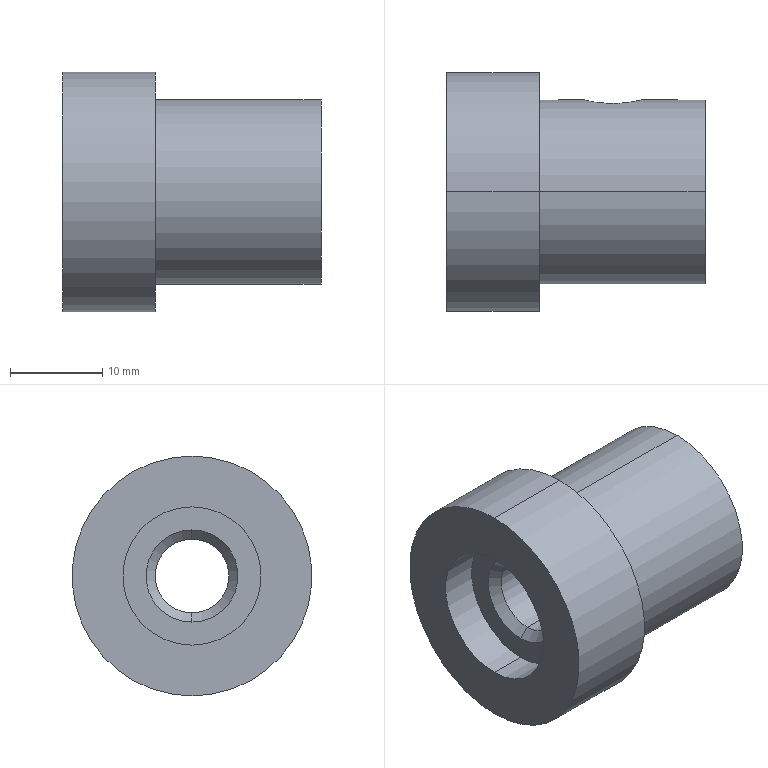Component | SolidWorks | LongAxisUpperSleeve-1 | 1 solid | 18 faces | box 28 x 26 x 26 mm | volume 8975 mm3 | cylinder 10 | cone 4 | plane 4 | commonest cylinder face diameters 3.2 x2 26 x2 20 x2 8 x2 15 x2 | material 5154-O, Bar (SS)
STEP:
#1=COLOUR_RGB('',0.7922,0.8196,0.9333);
#2=FILL_AREA_STYLE_COLOUR('',#1);
#3=FILL_AREA_STYLE('',(#2));
#4=SURFACE_STYLE_FILL_AREA(#3);
#5=SURFACE_SIDE_STYLE('',(#4));
#6=SURFACE_STYLE_USAGE(.BOTH.,#5);
#7=PRESENTATION_STYLE_ASSIGNMENT((#6));
#8=CARTESIAN_POINT('',(3.546,0.7394,13.677));
#9=VERTEX_POINT('',#8);
#10=CARTESIAN_POINT('',(3.546,0.7394,13.803));
#11=VERTEX_POINT('',#10);
#12=CARTESIAN_POINT('',(3.546,0.7394,13.677));
#13=CARTESIAN_POINT('',(3.542,0.7394,13.677));
#14=CARTESIAN_POINT('',(3.537,0.7396,13.678));
#15=CARTESIAN_POINT('',(3.529,0.7403,13.679));
#16=CARTESIAN_POINT('',(3.525,0.7408,13.68));
#17=CARTESIAN_POINT('',(3.514,0.7427,13.685));
#18=CARTESIAN_POINT('',(3.507,0.7444,13.69));
#19=CARTESIAN_POINT('',(3.498,0.747,13.699));
#20=CARTESIAN_POINT('',(3.496,0.7478,13.702));
#21=CARTESIAN_POINT('',(3.491,0.7494,13.708));
#22=CARTESIAN_POINT('',(3.489,0.7501,13.712));
#23=CARTESIAN_POINT('',(3.486,0.7513,13.72));
#24=CARTESIAN_POINT('',(3.485,0.7518,13.724));
#25=CARTESIAN_POINT('',(3.483,0.7524,13.732));
#26=CARTESIAN_POINT('',(3.483,0.7526,13.736));
#27=CARTESIAN_POINT('',(3.483,0.7526,13.748));
#28=CARTESIAN_POINT('',(3.484,0.7519,13.757));
#29=CARTESIAN_POINT('',(3.489,0.7501,13.768));
#30=CARTESIAN_POINT('',(3.491,0.7494,13.772));
#31=CARTESIAN_POINT('',(3.496,0.7478,13.779));
#32=CARTESIAN_POINT('',(3.498,0.747,13.782));
#33=CARTESIAN_POINT('',(3.504,0.7453,13.788));
#34=CARTESIAN_POINT('',(3.507,0.7444,13.79));
#35=CARTESIAN_POINT('',(3.514,0.7428,13.795));
#36=CARTESIAN_POINT('',(3.518,0.7421,13.797));
#37=CARTESIAN_POINT('',(3.529,0.7402,13.801));
#38=CARTESIAN_POINT('',(3.537,0.7394,13.803));
#39=CARTESIAN_POINT('',(3.546,0.7394,13.803));
#40=B_SPLINE_CURVE_WITH_KNOTS('',3,(#12,#13,#14,#15,#16,#17,#18,#19,#20,#21,#22,#23,#24,#25,#26,#27,#28,#29,#30,#31,#32,#33,#34,#35,#36,#37,#38,#39),.UNSPECIFIED.,.F.,.F.,(4,2,2,2,2,2,2,2,2,2,2,2,2,4),(0.005056,0.005371,0.005687,0.006318,0.006634,0.00695,0.007265,0.007581,0.008212,0.008528,0.008844,0.009159,0.009475,0.01011),.UNSPECIFIED.);
#41=EDGE_CURVE('',#9,#11,#40,.T.);
#42=ORIENTED_EDGE('',*,*,#41,.F.);
#43=CARTESIAN_POINT('',(3.546,0.9258,13.677));
#44=VERTEX_POINT('',#43);
#45=CARTESIAN_POINT('',(3.546,0.9888,13.677));
#46=DIRECTION('',(0.,1.,0.));
#47=VECTOR('',#46,39.37);
#48=LINE('',#45,#47);
#49=EDGE_CURVE('',#9,#44,#48,.T.);
#50=ORIENTED_EDGE('',*,*,#49,.T.);
#51=CARTESIAN_POINT('',(3.546,0.9258,13.803));
#52=VERTEX_POINT('',#51);
#53=CARTESIAN_POINT('',(3.546,0.9258,13.74));
#54=DIRECTION('',(0.,1.,0.));
#55=DIRECTION('',(0.,0.,1.));
#56=AXIS2_PLACEMENT_3D('',#53,#54,#55);
#57=CIRCLE('',#56,0.06299);
#58=EDGE_CURVE('',#44,#52,#57,.T.);
#59=ORIENTED_EDGE('',*,*,#58,.T.);
#60=CARTESIAN_POINT('',(3.546,0.9888,13.803));
#61=DIRECTION('',(0.,1.,0.));
#62=VECTOR('',#61,39.37);
#63=LINE('',#60,#62);
#64=EDGE_CURVE('',#11,#52,#63,.T.);
#65=ORIENTED_EDGE('',*,*,#64,.F.);
#66=EDGE_LOOP('',(#42,#50,#59,#65));
#67=FACE_OUTER_BOUND('',#66,.T.);
#68=CARTESIAN_POINT('',(3.546,0.9888,13.74));
#69=DIRECTION('',(0.,1.,0.));
#70=DIRECTION('',(0.,0.,1.));
#71=AXIS2_PLACEMENT_3D('',#68,#69,#70);
#72=CYLINDRICAL_SURFACE('',#71,0.06299);
#73=ADVANCED_FACE('',(#67),#72,.F.);
#74=ORIENTED_EDGE('',*,*,#58,.F.);
#75=CARTESIAN_POINT('',(3.546,0.9731,13.63));
#76=VERTEX_POINT('',#75);
#77=CARTESIAN_POINT('',(3.546,0.9888,13.614));
#78=DIRECTION('',(0.,0.7071,-0.7071));
#79=VECTOR('',#78,39.37);
#80=LINE('',#77,#79);
#81=EDGE_CURVE('',#44,#76,#80,.T.);
#82=ORIENTED_EDGE('',*,*,#81,.T.);
#83=CARTESIAN_POINT('',(3.546,0.9731,13.85));
#84=VERTEX_POINT('',#83);
#85=CARTESIAN_POINT('',(3.546,0.9731,13.85));
#86=CARTESIAN_POINT('',(3.53,0.9731,13.85));
#87=CARTESIAN_POINT('',(3.515,0.9738,13.848));
#88=CARTESIAN_POINT('',(3.493,0.9759,13.84));
#89=CARTESIAN_POINT('',(3.486,0.9767,13.837));
#90=CARTESIAN_POINT('',(3.472,0.9785,13.83));
#91=CARTESIAN_POINT('',(3.466,0.9795,13.825));
#92=CARTESIAN_POINT('',(3.454,0.9815,13.816));
#93=CARTESIAN_POINT('',(3.448,0.9825,13.81));
#94=CARTESIAN_POINT('',(3.439,0.9845,13.798));
#95=CARTESIAN_POINT('',(3.434,0.9854,13.792));
#96=CARTESIAN_POINT('',(3.427,0.987,13.778));
#97=CARTESIAN_POINT('',(3.424,0.9877,13.771));
#98=CARTESIAN_POINT('',(3.421,0.9886,13.756));
#99=CARTESIAN_POINT('',(3.42,0.9888,13.748));
#100=CARTESIAN_POINT('',(3.42,0.9888,13.732));
#101=CARTESIAN_POINT('',(3.421,0.9886,13.725));
#102=CARTESIAN_POINT('',(3.424,0.9877,13.71));
#103=CARTESIAN_POINT('',(3.427,0.987,13.702));
#104=CARTESIAN_POINT('',(3.434,0.9855,13.689));
#105=CARTESIAN_POINT('',(3.439,0.9845,13.682));
#106=CARTESIAN_POINT('',(3.448,0.9826,13.67));
#107=CARTESIAN_POINT('',(3.454,0.9815,13.665));
#108=CARTESIAN_POINT('',(3.472,0.9784,13.65));
#109=CARTESIAN_POINT('',(3.485,0.9765,13.643));
#110=CARTESIAN_POINT('',(3.507,0.9745,13.635));
#111=CARTESIAN_POINT('',(3.515,0.974,13.633));
#112=CARTESIAN_POINT('',(3.53,0.9732,13.631));
#113=CARTESIAN_POINT('',(3.538,0.9731,13.63));
#114=CARTESIAN_POINT('',(3.546,0.9731,13.63));
#115=B_SPLINE_CURVE_WITH_KNOTS('',3,(#85,#86,#87,#88,#89,#90,#91,#92,#93,#94,#95,#96,#97,#98,#99,#100,#101,#102,#103,#104,#105,#106,#107,#108,#109,#110,#111,#112,#113,#114),.UNSPECIFIED.,.F.,.F.,(4,2,2,2,2,2,2,2,2,2,2,2,2,2,4),(0.01171,0.01289,0.01348,0.01406,0.01465,0.01524,0.01583,0.01642,0.017,0.01759,0.01818,0.01877,0.01994,0.02053,0.02112),.UNSPECIFIED.);
#116=EDGE_CURVE('',#84,#76,#115,.T.);
#117=ORIENTED_EDGE('',*,*,#116,.F.);
#118=CARTESIAN_POINT('',(3.546,0.9888,13.866));
#119=DIRECTION('',(0.,0.7071,0.7071));
#120=VECTOR('',#119,39.37);
#121=LINE('',#118,#120);
#122=EDGE_CURVE('',#52,#84,#121,.T.);
#123=ORIENTED_EDGE('',*,*,#122,.F.);
#124=EDGE_LOOP('',(#74,#82,#117,#123));
#125=FACE_OUTER_BOUND('',#124,.T.);
#126=CARTESIAN_POINT('',(3.546,0.9888,13.74));
#127=DIRECTION('',(0.,1.,0.));
#128=DIRECTION('',(0.,0.,1.));
#129=AXIS2_PLACEMENT_3D('',#126,#127,#128);
#130=CONICAL_SURFACE('',#129,0.126,0.7854);
#131=ADVANCED_FACE('',(#125),#130,.F.);
#132=CARTESIAN_POINT('',(3.231,0.5951,14.252));
#133=VERTEX_POINT('',#132);
#134=CARTESIAN_POINT('',(3.231,0.5951,13.228));
#135=VERTEX_POINT('',#134);
#136=CARTESIAN_POINT('',(3.231,0.5951,13.74));
#137=DIRECTION('',(-1.,0.,0.));
#138=DIRECTION('',(0.,0.,1.));
#139=AXIS2_PLACEMENT_3D('',#136,#137,#138);
#140=CIRCLE('',#139,0.5118);
#141=EDGE_CURVE('',#133,#135,#140,.T.);
#142=ORIENTED_EDGE('',*,*,#141,.T.);
#143=CARTESIAN_POINT('',(2.837,0.5951,13.228));
#144=VERTEX_POINT('',#143);
#145=CARTESIAN_POINT('',(-0.1135,0.5951,13.228));
#146=DIRECTION('',(-1.,0.,0.));
#147=VECTOR('',#146,39.37);
#148=LINE('',#145,#147);
#149=EDGE_CURVE('',#135,#144,#148,.T.);
#150=ORIENTED_EDGE('',*,*,#149,.T.);
#151=CARTESIAN_POINT('',(2.837,0.5951,14.252));
#152=VERTEX_POINT('',#151);
#153=CARTESIAN_POINT('',(2.837,0.5951,13.74));
#154=DIRECTION('',(-1.,0.,0.));
#155=DIRECTION('',(0.,0.,1.));
#156=AXIS2_PLACEMENT_3D('',#153,#154,#155);
#157=CIRCLE('',#156,0.5118);
#158=EDGE_CURVE('',#152,#144,#157,.T.);
#159=ORIENTED_EDGE('',*,*,#158,.F.);
#160=CARTESIAN_POINT('',(-0.1135,0.5951,14.252));
#161=DIRECTION('',(-1.,0.,0.));
#162=VECTOR('',#161,39.37);
#163=LINE('',#160,#162);
#164=EDGE_CURVE('',#133,#152,#163,.T.);
#165=ORIENTED_EDGE('',*,*,#164,.F.);
#166=EDGE_LOOP('',(#142,#150,#159,#165));
#167=FACE_OUTER_BOUND('',#166,.T.);
#168=CARTESIAN_POINT('',(-0.1135,0.5951,13.74));
#169=DIRECTION('',(-1.,0.,0.));
#170=DIRECTION('',(0.,0.,1.));
#171=AXIS2_PLACEMENT_3D('',#168,#169,#170);
#172=CYLINDRICAL_SURFACE('',#171,0.5118);
#173=ADVANCED_FACE('',(#167),#172,.T.);
#174=ORIENTED_EDGE('',*,*,#116,.T.);
#175=CARTESIAN_POINT('',(3.546,0.9731,13.63));
#176=CARTESIAN_POINT('',(3.554,0.9731,13.63));
#177=CARTESIAN_POINT('',(3.561,0.9732,13.631));
#178=CARTESIAN_POINT('',(3.576,0.974,13.633));
#179=CARTESIAN_POINT('',(3.584,0.9745,13.635));
#180=CARTESIAN_POINT('',(3.599,0.9759,13.64));
#181=CARTESIAN_POINT('',(3.606,0.9767,13.643));
#182=CARTESIAN_POINT('',(3.619,0.9785,13.65));
#183=CARTESIAN_POINT('',(3.626,0.9795,13.655));
#184=CARTESIAN_POINT('',(3.638,0.9815,13.665));
#185=CARTESIAN_POINT('',(3.643,0.9825,13.67));
#186=CARTESIAN_POINT('',(3.653,0.9845,13.682));
#187=CARTESIAN_POINT('',(3.657,0.9854,13.688));
#188=CARTESIAN_POINT('',(3.664,0.987,13.702));
#189=CARTESIAN_POINT('',(3.667,0.9877,13.709));
#190=CARTESIAN_POINT('',(3.671,0.9886,13.724));
#191=CARTESIAN_POINT('',(3.672,0.9888,13.732));
#192=CARTESIAN_POINT('',(3.672,0.9888,13.748));
#193=CARTESIAN_POINT('',(3.671,0.9886,13.755));
#194=CARTESIAN_POINT('',(3.667,0.9877,13.77));
#195=CARTESIAN_POINT('',(3.664,0.9871,13.778));
#196=CARTESIAN_POINT('',(3.654,0.9847,13.798));
#197=CARTESIAN_POINT('',(3.644,0.9826,13.811));
#198=CARTESIAN_POINT('',(3.626,0.9795,13.825));
#199=CARTESIAN_POINT('',(3.619,0.9785,13.83));
#200=CARTESIAN_POINT('',(3.606,0.9767,13.837));
#201=CARTESIAN_POINT('',(3.599,0.9759,13.84));
#202=CARTESIAN_POINT('',(3.584,0.9745,13.845));
#203=CARTESIAN_POINT('',(3.577,0.974,13.847));
#204=CARTESIAN_POINT('',(3.561,0.9732,13.85));
#205=CARTESIAN_POINT('',(3.553,0.9731,13.85));
#206=CARTESIAN_POINT('',(3.546,0.9731,13.85));
#207=B_SPLINE_CURVE_WITH_KNOTS('',3,(#175,#176,#177,#178,#179,#180,#181,#182,#183,#184,#185,#186,#187,#188,#189,#190,#191,#192,#193,#194,#195,#196,#197,#198,#199,#200,#201,#202,#203,#204,#205,#206),.UNSPECIFIED.,.F.,.F.,(4,2,2,2,2,2,2,2,2,2,2,2,2,2,2,4),(0.0023,0.002888,0.003477,0.004065,0.004653,0.005242,0.00583,0.006419,0.007007,0.007595,0.008184,0.00936,0.009949,0.01054,0.01113,0.01171),.UNSPECIFIED.);
#208=EDGE_CURVE('',#76,#84,#207,.T.);
#209=ORIENTED_EDGE('',*,*,#208,.T.);
#210=EDGE_LOOP('',(#174,#209));
#211=FACE_BOUND('',#210,.T.);
#212=CARTESIAN_POINT('',(3.939,0.5951,14.134));
#213=VERTEX_POINT('',#212);
#214=CARTESIAN_POINT('',(3.939,0.5951,13.346));
#215=VERTEX_POINT('',#214);
#216=CARTESIAN_POINT('',(3.939,0.5951,13.74));
#217=DIRECTION('',(-1.,0.,0.));
#218=DIRECTION('',(0.,0.,1.));
#219=AXIS2_PLACEMENT_3D('',#216,#217,#218);
#220=CIRCLE('',#219,0.3937);
#221=EDGE_CURVE('',#213,#215,#220,.T.);
#222=ORIENTED_EDGE('',*,*,#221,.T.);
#223=CARTESIAN_POINT('',(3.231,0.5951,13.346));
#224=VERTEX_POINT('',#223);
#225=CARTESIAN_POINT('',(-0.1135,0.5951,13.346));
#226=DIRECTION('',(-1.,0.,0.));
#227=VECTOR('',#226,39.37);
#228=LINE('',#225,#227);
#229=EDGE_CURVE('',#215,#224,#228,.T.);
#230=ORIENTED_EDGE('',*,*,#229,.T.);
#231=CARTESIAN_POINT('',(3.231,0.5951,14.134));
#232=VERTEX_POINT('',#231);
#233=CARTESIAN_POINT('',(3.231,0.5951,13.74));
#234=DIRECTION('',(-1.,0.,0.));
#235=DIRECTION('',(0.,0.,1.));
#236=AXIS2_PLACEMENT_3D('',#233,#234,#235);
#237=CIRCLE('',#236,0.3937);
#238=EDGE_CURVE('',#232,#224,#237,.T.);
#239=ORIENTED_EDGE('',*,*,#238,.F.);
#240=CARTESIAN_POINT('',(-0.1135,0.5951,14.134));
#241=DIRECTION('',(-1.,0.,0.));
#242=VECTOR('',#241,39.37);
#243=LINE('',#240,#242);
#244=EDGE_CURVE('',#213,#232,#243,.T.);
#245=ORIENTED_EDGE('',*,*,#244,.F.);
#246=EDGE_LOOP('',(#222,#230,#239,#245));
#247=FACE_OUTER_BOUND('',#246,.T.);
#248=CARTESIAN_POINT('',(-0.1135,0.5951,13.74));
#249=DIRECTION('',(-1.,0.,0.));
#250=DIRECTION('',(0.,0.,1.));
#251=AXIS2_PLACEMENT_3D('',#248,#249,#250);
#252=CYLINDRICAL_SURFACE('',#251,0.3937);
#253=ADVANCED_FACE('',(#211,#247),#252,.T.);
#254=CARTESIAN_POINT('',(3.939,0.5951,13.583));
#255=VERTEX_POINT('',#254);
#256=CARTESIAN_POINT('',(3.939,0.5951,13.898));
#257=VERTEX_POINT('',#256);
#258=CARTESIAN_POINT('',(3.939,0.5951,13.74));
#259=DIRECTION('',(-1.,0.,0.));
#260=DIRECTION('',(0.,0.,1.));
#261=AXIS2_PLACEMENT_3D('',#258,#259,#260);
#262=CIRCLE('',#261,0.1575);
#263=EDGE_CURVE('',#255,#257,#262,.T.);
#264=ORIENTED_EDGE('',*,*,#263,.F.);
#265=CARTESIAN_POINT('',(3.034,0.5951,13.583));
#266=VERTEX_POINT('',#265);
#267=CARTESIAN_POINT('',(-0.1135,0.5951,13.583));
#268=DIRECTION('',(-1.,0.,0.));
#269=VECTOR('',#268,39.37);
#270=LINE('',#267,#269);
#271=EDGE_CURVE('',#255,#266,#270,.T.);
#272=ORIENTED_EDGE('',*,*,#271,.T.);
#273=CARTESIAN_POINT('',(3.034,0.5951,13.898));
#274=VERTEX_POINT('',#273);
#275=CARTESIAN_POINT('',(3.034,0.5951,13.74));
#276=DIRECTION('',(-1.,0.,0.));
#277=DIRECTION('',(0.,0.,1.));
#278=AXIS2_PLACEMENT_3D('',#275,#276,#277);
#279=CIRCLE('',#278,0.1575);
#280=EDGE_CURVE('',#266,#274,#279,.T.);
#281=ORIENTED_EDGE('',*,*,#280,.T.);
#282=CARTESIAN_POINT('',(-0.1135,0.5951,13.898));
#283=DIRECTION('',(-1.,0.,0.));
#284=VECTOR('',#283,39.37);
#285=LINE('',#282,#284);
#286=EDGE_CURVE('',#257,#274,#285,.T.);
#287=ORIENTED_EDGE('',*,*,#286,.F.);
#288=EDGE_LOOP('',(#264,#272,#281,#287));
#289=FACE_OUTER_BOUND('',#288,.T.);
#290=CARTESIAN_POINT('',(-0.1135,0.5951,13.74));
#291=DIRECTION('',(-1.,0.,0.));
#292=DIRECTION('',(0.,0.,1.));
#293=AXIS2_PLACEMENT_3D('',#290,#291,#292);
#294=CYLINDRICAL_SURFACE('',#293,0.1575);
#295=ADVANCED_FACE('',(#289),#294,.F.);
#296=ORIENTED_EDGE('',*,*,#280,.F.);
#297=CARTESIAN_POINT('',(2.995,0.5951,13.543));
#298=VERTEX_POINT('',#297);
#299=CARTESIAN_POINT('',(2.995,0.5951,13.543));
#300=DIRECTION('',(-0.7071,0.,-0.7071));
#301=VECTOR('',#300,39.37);
#302=LINE('',#299,#301);
#303=EDGE_CURVE('',#266,#298,#302,.T.);
#304=ORIENTED_EDGE('',*,*,#303,.T.);
#305=CARTESIAN_POINT('',(2.995,0.5951,13.937));
#306=VERTEX_POINT('',#305);
#307=CARTESIAN_POINT('',(2.995,0.5951,13.74));
#308=DIRECTION('',(-1.,0.,0.));
#309=DIRECTION('',(0.,0.,1.));
#310=AXIS2_PLACEMENT_3D('',#307,#308,#309);
#311=CIRCLE('',#310,0.1969);
#312=EDGE_CURVE('',#298,#306,#311,.T.);
#313=ORIENTED_EDGE('',*,*,#312,.T.);
#314=CARTESIAN_POINT('',(2.995,0.5951,13.937));
#315=DIRECTION('',(-0.7071,0.,0.7071));
#316=VECTOR('',#315,39.37);
#317=LINE('',#314,#316);
#318=EDGE_CURVE('',#274,#306,#317,.T.);
#319=ORIENTED_EDGE('',*,*,#318,.F.);
#320=EDGE_LOOP('',(#296,#304,#313,#319));
#321=FACE_OUTER_BOUND('',#320,.T.);
#322=CARTESIAN_POINT('',(2.995,0.5951,13.74));
#323=DIRECTION('',(-1.,0.,0.));
#324=DIRECTION('',(0.,0.,1.));
#325=AXIS2_PLACEMENT_3D('',#322,#323,#324);
#326=CONICAL_SURFACE('',#325,0.1969,0.7854);
#327=ADVANCED_FACE('',(#321),#326,.F.);
#328=CARTESIAN_POINT('',(2.995,0.5951,13.445));
#329=VERTEX_POINT('',#328);
#330=CARTESIAN_POINT('',(2.995,0.5951,14.035));
#331=VERTEX_POINT('',#330);
#332=CARTESIAN_POINT('',(2.995,0.5951,13.74));
#333=DIRECTION('',(-1.,0.,0.));
#334=DIRECTION('',(0.,0.,1.));
#335=AXIS2_PLACEMENT_3D('',#332,#333,#334);
#336=CIRCLE('',#335,0.2953);
#337=EDGE_CURVE('',#329,#331,#336,.T.);
#338=ORIENTED_EDGE('',*,*,#337,.F.);
#339=CARTESIAN_POINT('',(2.837,0.5951,13.445));
#340=VERTEX_POINT('',#339);
#341=CARTESIAN_POINT('',(-0.1135,0.5951,13.445));
#342=DIRECTION('',(-1.,0.,0.));
#343=VECTOR('',#342,39.37);
#344=LINE('',#341,#343);
#345=EDGE_CURVE('',#329,#340,#344,.T.);
#346=ORIENTED_EDGE('',*,*,#345,.T.);
#347=CARTESIAN_POINT('',(2.837,0.5951,14.035));
#348=VERTEX_POINT('',#347);
#349=CARTESIAN_POINT('',(2.837,0.5951,13.74));
#350=DIRECTION('',(-1.,0.,0.));
#351=DIRECTION('',(0.,0.,1.));
#352=AXIS2_PLACEMENT_3D('',#349,#350,#351);
#353=CIRCLE('',#352,0.2953);
#354=EDGE_CURVE('',#340,#348,#353,.T.);
#355=ORIENTED_EDGE('',*,*,#354,.T.);
#356=CARTESIAN_POINT('',(-0.1135,0.5951,14.035));
#357=DIRECTION('',(-1.,0.,0.));
#358=VECTOR('',#357,39.37);
#359=LINE('',#356,#358);
#360=EDGE_CURVE('',#331,#348,#359,.T.);
#361=ORIENTED_EDGE('',*,*,#360,.F.);
#362=EDGE_LOOP('',(#338,#346,#355,#361));
#363=FACE_OUTER_BOUND('',#362,.T.);
#364=CARTESIAN_POINT('',(-0.1135,0.5951,13.74));
#365=DIRECTION('',(-1.,0.,0.));
#366=DIRECTION('',(0.,0.,1.));
#367=AXIS2_PLACEMENT_3D('',#364,#365,#366);
#368=CYLINDRICAL_SURFACE('',#367,0.2953);
#369=ADVANCED_FACE('',(#363),#368,.F.);
#370=CARTESIAN_POINT('',(2.837,0.5951,13.74));
#371=DIRECTION('',(-1.,0.,0.));
#372=DIRECTION('',(0.,0.,1.));
#373=AXIS2_PLACEMENT_3D('',#370,#371,#372);
#374=CIRCLE('',#373,0.2953);
#375=EDGE_CURVE('',#348,#340,#374,.T.);
#376=ORIENTED_EDGE('',*,*,#375,.F.);
#377=ORIENTED_EDGE('',*,*,#354,.F.);
#378=EDGE_LOOP('',(#376,#377));
#379=FACE_BOUND('',#378,.T.);
#380=ORIENTED_EDGE('',*,*,#158,.T.);
#381=CARTESIAN_POINT('',(2.837,0.5951,13.74));
#382=DIRECTION('',(-1.,0.,0.));
#383=DIRECTION('',(0.,0.,1.));
#384=AXIS2_PLACEMENT_3D('',#381,#382,#383);
#385=CIRCLE('',#384,0.5118);
#386=EDGE_CURVE('',#144,#152,#385,.T.);
#387=ORIENTED_EDGE('',*,*,#386,.T.);
#388=EDGE_LOOP('',(#380,#387));
#389=FACE_OUTER_BOUND('',#388,.T.);
#390=CARTESIAN_POINT('',(2.837,1.107,13.74));
#391=DIRECTION('',(1.,0.,0.));
#392=DIRECTION('',(0.,0.,-1.));
#393=AXIS2_PLACEMENT_3D('',#390,#391,#392);
#394=PLANE('',#393);
#395=ADVANCED_FACE('',(#379,#389),#394,.F.);
#396=ORIENTED_EDGE('',*,*,#345,.F.);
#397=CARTESIAN_POINT('',(2.995,0.5951,13.74));
#398=DIRECTION('',(-1.,0.,0.));
#399=DIRECTION('',(0.,0.,1.));
#400=AXIS2_PLACEMENT_3D('',#397,#398,#399);
#401=CIRCLE('',#400,0.2953);
#402=EDGE_CURVE('',#331,#329,#401,.T.);
#403=ORIENTED_EDGE('',*,*,#402,.F.);
#404=ORIENTED_EDGE('',*,*,#360,.T.);
#405=ORIENTED_EDGE('',*,*,#375,.T.);
#406=EDGE_LOOP('',(#396,#403,#404,#405));
#407=FACE_OUTER_BOUND('',#406,.T.);
#408=CARTESIAN_POINT('',(-0.1135,0.5951,13.74));
#409=DIRECTION('',(-1.,0.,0.));
#410=DIRECTION('',(0.,0.,1.));
#411=AXIS2_PLACEMENT_3D('',#408,#409,#410);
#412=CYLINDRICAL_SURFACE('',#411,0.2953);
#413=ADVANCED_FACE('',(#407),#412,.F.);
#414=CARTESIAN_POINT('',(2.995,0.5951,13.74));
#415=DIRECTION('',(-1.,0.,0.));
#416=DIRECTION('',(0.,0.,1.));
#417=AXIS2_PLACEMENT_3D('',#414,#415,#416);
#418=CIRCLE('',#417,0.1969);
#419=EDGE_CURVE('',#306,#298,#418,.T.);
#420=ORIENTED_EDGE('',*,*,#419,.F.);
#421=ORIENTED_EDGE('',*,*,#312,.F.);
#422=EDGE_LOOP('',(#420,#421));
#423=FACE_BOUND('',#422,.T.);
#424=ORIENTED_EDGE('',*,*,#402,.T.);
#425=ORIENTED_EDGE('',*,*,#337,.T.);
#426=EDGE_LOOP('',(#424,#425));
#427=FACE_OUTER_BOUND('',#426,.T.);
#428=CARTESIAN_POINT('',(2.995,0.8904,13.74));
#429=DIRECTION('',(1.,0.,0.));
#430=DIRECTION('',(0.,0.,-1.));
#431=AXIS2_PLACEMENT_3D('',#428,#429,#430);
#432=PLANE('',#431);
#433=ADVANCED_FACE('',(#423,#427),#432,.F.);
#434=ORIENTED_EDGE('',*,*,#303,.F.);
#435=CARTESIAN_POINT('',(3.034,0.5951,13.74));
#436=DIRECTION('',(-1.,0.,0.));
#437=DIRECTION('',(0.,0.,1.));
#438=AXIS2_PLACEMENT_3D('',#435,#436,#437);
#439=CIRCLE('',#438,0.1575);
#440=EDGE_CURVE('',#274,#266,#439,.T.);
#441=ORIENTED_EDGE('',*,*,#440,.F.);
#442=ORIENTED_EDGE('',*,*,#318,.T.);
#443=ORIENTED_EDGE('',*,*,#419,.T.);
#444=EDGE_LOOP('',(#434,#441,#442,#443));
#445=FACE_OUTER_BOUND('',#444,.T.);
#446=CARTESIAN_POINT('',(2.995,0.5951,13.74));
#447=DIRECTION('',(-1.,0.,0.));
#448=DIRECTION('',(0.,0.,1.));
#449=AXIS2_PLACEMENT_3D('',#446,#447,#448);
#450=CONICAL_SURFACE('',#449,0.1969,0.7854);
#451=ADVANCED_FACE('',(#445),#450,.F.);
#452=ORIENTED_EDGE('',*,*,#271,.F.);
#453=CARTESIAN_POINT('',(3.939,0.5951,13.74));
#454=DIRECTION('',(-1.,0.,0.));
#455=DIRECTION('',(0.,0.,1.));
#456=AXIS2_PLACEMENT_3D('',#453,#454,#455);
#457=CIRCLE('',#456,0.1575);
#458=EDGE_CURVE('',#257,#255,#457,.T.);
#459=ORIENTED_EDGE('',*,*,#458,.F.);
#460=ORIENTED_EDGE('',*,*,#286,.T.);
#461=ORIENTED_EDGE('',*,*,#440,.T.);
#462=EDGE_LOOP('',(#452,#459,#460,#461));
#463=FACE_OUTER_BOUND('',#462,.T.);
#464=CARTESIAN_POINT('',(3.546,0.7394,13.803));
#465=CARTESIAN_POINT('',(3.55,0.7394,13.803));
#466=CARTESIAN_POINT('',(3.554,0.7396,13.803));
#467=CARTESIAN_POINT('',(3.562,0.7403,13.801));
#468=CARTESIAN_POINT('',(3.566,0.7408,13.8));
#469=CARTESIAN_POINT('',(3.578,0.7427,13.795));
#470=CARTESIAN_POINT('',(3.585,0.7445,13.79));
#471=CARTESIAN_POINT('',(3.596,0.7479,13.779));
#472=CARTESIAN_POINT('',(3.601,0.7495,13.772));
#473=CARTESIAN_POINT('',(3.605,0.7513,13.761));
#474=CARTESIAN_POINT('',(3.607,0.7518,13.757));
#475=CARTESIAN_POINT('',(3.608,0.7524,13.748));
#476=CARTESIAN_POINT('',(3.609,0.7526,13.744));
#477=CARTESIAN_POINT('',(3.609,0.7526,13.736));
#478=CARTESIAN_POINT('',(3.608,0.7524,13.732));
#479=CARTESIAN_POINT('',(3.607,0.7518,13.724));
#480=CARTESIAN_POINT('',(3.605,0.7513,13.72));
#481=CARTESIAN_POINT('',(3.602,0.7501,13.712));
#482=CARTESIAN_POINT('',(3.6,0.7494,13.708));
#483=CARTESIAN_POINT('',(3.596,0.7478,13.702));
#484=CARTESIAN_POINT('',(3.593,0.747,13.698));
#485=CARTESIAN_POINT('',(3.587,0.7453,13.693));
#486=CARTESIAN_POINT('',(3.584,0.7444,13.69));
#487=CARTESIAN_POINT('',(3.577,0.7428,13.686));
#488=CARTESIAN_POINT('',(3.574,0.7421,13.684));
#489=CARTESIAN_POINT('',(3.562,0.7402,13.679));
#490=CARTESIAN_POINT('',(3.554,0.7394,13.677));
#491=CARTESIAN_POINT('',(3.546,0.7394,13.677));
#492=B_SPLINE_CURVE_WITH_KNOTS('',3,(#464,#465,#466,#467,#468,#469,#470,#471,#472,#473,#474,#475,#476,#477,#478,#479,#480,#481,#482,#483,#484,#485,#486,#487,#488,#489,#490,#491),.UNSPECIFIED.,.F.,.F.,(4,2,2,2,2,2,2,2,2,2,2,2,2,4),(0.,0.000316,0.0006319,0.001264,0.001896,0.002212,0.002528,0.002844,0.00316,0.003476,0.003792,0.004108,0.004424,0.005056),.UNSPECIFIED.);
#493=EDGE_CURVE('',#11,#9,#492,.T.);
#494=ORIENTED_EDGE('',*,*,#493,.T.);
#495=ORIENTED_EDGE('',*,*,#41,.T.);
#496=EDGE_LOOP('',(#494,#495));
#497=FACE_BOUND('',#496,.T.);
#498=CARTESIAN_POINT('',(-0.1135,0.5951,13.74));
#499=DIRECTION('',(-1.,0.,0.));
#500=DIRECTION('',(0.,0.,1.));
#501=AXIS2_PLACEMENT_3D('',#498,#499,#500);
#502=CYLINDRICAL_SURFACE('',#501,0.1575);
#503=ADVANCED_FACE('',(#463,#497),#502,.F.);
#504=ORIENTED_EDGE('',*,*,#221,.F.);
#505=CARTESIAN_POINT('',(3.939,0.5951,13.74));
#506=DIRECTION('',(-1.,0.,0.));
#507=DIRECTION('',(0.,0.,1.));
#508=AXIS2_PLACEMENT_3D('',#505,#506,#507);
#509=CIRCLE('',#508,0.3937);
#510=EDGE_CURVE('',#215,#213,#509,.T.);
#511=ORIENTED_EDGE('',*,*,#510,.F.);
#512=EDGE_LOOP('',(#504,#511));
#513=FACE_OUTER_BOUND('',#512,.T.);
#514=ORIENTED_EDGE('',*,*,#458,.T.);
#515=ORIENTED_EDGE('',*,*,#263,.T.);
#516=EDGE_LOOP('',(#514,#515));
#517=FACE_BOUND('',#516,.T.);
#518=CARTESIAN_POINT('',(3.939,0.9888,13.74));
#519=DIRECTION('',(-1.,0.,0.));
#520=DIRECTION('',(0.,0.,1.));
#521=AXIS2_PLACEMENT_3D('',#518,#519,#520);
#522=PLANE('',#521);
#523=ADVANCED_FACE('',(#513,#517),#522,.F.);
#524=ORIENTED_EDGE('',*,*,#229,.F.);
#525=ORIENTED_EDGE('',*,*,#510,.T.);
#526=ORIENTED_EDGE('',*,*,#244,.T.);
#527=CARTESIAN_POINT('',(3.231,0.5951,13.74));
#528=DIRECTION('',(-1.,0.,0.));
#529=DIRECTION('',(0.,0.,1.));
#530=AXIS2_PLACEMENT_3D('',#527,#528,#529);
#531=CIRCLE('',#530,0.3937);
#532=EDGE_CURVE('',#224,#232,#531,.T.);
#533=ORIENTED_EDGE('',*,*,#532,.F.);
#534=EDGE_LOOP('',(#524,#525,#526,#533));
#535=FACE_OUTER_BOUND('',#534,.T.);
#536=CARTESIAN_POINT('',(-0.1135,0.5951,13.74));
#537=DIRECTION('',(-1.,0.,0.));
#538=DIRECTION('',(0.,0.,1.));
#539=AXIS2_PLACEMENT_3D('',#536,#537,#538);
#540=CYLINDRICAL_SURFACE('',#539,0.3937);
#541=ADVANCED_FACE('',(#535),#540,.T.);
#542=ORIENTED_EDGE('',*,*,#141,.F.);
#543=CARTESIAN_POINT('',(3.231,0.5951,13.74));
#544=DIRECTION('',(-1.,0.,0.));
#545=DIRECTION('',(0.,0.,1.));
#546=AXIS2_PLACEMENT_3D('',#543,#544,#545);
#547=CIRCLE('',#546,0.5118);
#548=EDGE_CURVE('',#135,#133,#547,.T.);
#549=ORIENTED_EDGE('',*,*,#548,.F.);
#550=EDGE_LOOP('',(#542,#549));
#551=FACE_OUTER_BOUND('',#550,.T.);
#552=ORIENTED_EDGE('',*,*,#238,.T.);
#553=ORIENTED_EDGE('',*,*,#532,.T.);
#554=EDGE_LOOP('',(#552,#553));
#555=FACE_BOUND('',#554,.T.);
#556=CARTESIAN_POINT('',(3.231,1.107,13.74));
#557=DIRECTION('',(-1.,0.,0.));
#558=DIRECTION('',(0.,0.,1.));
#559=AXIS2_PLACEMENT_3D('',#556,#557,#558);
#560=PLANE('',#559);
#561=ADVANCED_FACE('',(#551,#555),#560,.F.);
#562=ORIENTED_EDGE('',*,*,#149,.F.);
#563=ORIENTED_EDGE('',*,*,#548,.T.);
#564=ORIENTED_EDGE('',*,*,#164,.T.);
#565=ORIENTED_EDGE('',*,*,#386,.F.);
#566=EDGE_LOOP('',(#562,#563,#564,#565));
#567=FACE_OUTER_BOUND('',#566,.T.);
#568=CARTESIAN_POINT('',(-0.1135,0.5951,13.74));
#569=DIRECTION('',(-1.,0.,0.));
#570=DIRECTION('',(0.,0.,1.));
#571=AXIS2_PLACEMENT_3D('',#568,#569,#570);
#572=CYLINDRICAL_SURFACE('',#571,0.5118);
#573=ADVANCED_FACE('',(#567),#572,.T.);
#574=ORIENTED_EDGE('',*,*,#81,.F.);
#575=CARTESIAN_POINT('',(3.546,0.9258,13.74));
#576=DIRECTION('',(0.,1.,0.));
#577=DIRECTION('',(0.,0.,1.));
#578=AXIS2_PLACEMENT_3D('',#575,#576,#577);
#579=CIRCLE('',#578,0.06299);
#580=EDGE_CURVE('',#52,#44,#579,.T.);
#581=ORIENTED_EDGE('',*,*,#580,.F.);
#582=ORIENTED_EDGE('',*,*,#122,.T.);
#583=ORIENTED_EDGE('',*,*,#208,.F.);
#584=EDGE_LOOP('',(#574,#581,#582,#583));
#585=FACE_OUTER_BOUND('',#584,.T.);
#586=CARTESIAN_POINT('',(3.546,0.9888,13.74));
#587=DIRECTION('',(0.,1.,0.));
#588=DIRECTION('',(0.,0.,1.));
#589=AXIS2_PLACEMENT_3D('',#586,#587,#588);
#590=CONICAL_SURFACE('',#589,0.126,0.7854);
#591=ADVANCED_FACE('',(#585),#590,.F.);
#592=ORIENTED_EDGE('',*,*,#49,.F.);
#593=ORIENTED_EDGE('',*,*,#493,.F.);
#594=ORIENTED_EDGE('',*,*,#64,.T.);
#595=ORIENTED_EDGE('',*,*,#580,.T.);
#596=EDGE_LOOP('',(#592,#593,#594,#595));
#597=FACE_OUTER_BOUND('',#596,.T.);
#598=CARTESIAN_POINT('',(3.546,0.9888,13.74));
#599=DIRECTION('',(0.,1.,0.));
#600=DIRECTION('',(0.,0.,1.));
#601=AXIS2_PLACEMENT_3D('',#598,#599,#600);
#602=CYLINDRICAL_SURFACE('',#601,0.06299);
#603=ADVANCED_FACE('',(#597),#602,.F.);
#604=CLOSED_SHELL('',(#73,#131,#173,#253,#295,#327,#369,#395,#413,#433,#451,#503,#523,#541,#561,#573,#591,#603));
#605=MANIFOLD_SOLID_BREP('',#604);
#606=STYLED_ITEM('',(#7),#605);
#607=PRESENTATION_LAYER_ASSIGNMENT('','',(#606));
#608=CARTESIAN_POINT('',(0.,0.,0.));
#609=DIRECTION('',(0.,0.,1.));
#610=DIRECTION('',(1.,0.,0.));
#611=AXIS2_PLACEMENT_3D('',#608,#609,#610);
#612=(LENGTH_UNIT()NAMED_UNIT(*)SI_UNIT($,.METRE.));
#613=LENGTH_MEASURE_WITH_UNIT(LENGTH_MEASURE(0.0254),#612);
#614=DIMENSIONAL_EXPONENTS(1.,0.,0.,0.,0.,0.,0.);
#615=(CONVERSION_BASED_UNIT('',#613)LENGTH_UNIT()NAMED_UNIT(#614));
#616=UNCERTAINTY_MEASURE_WITH_UNIT(LENGTH_MEASURE(0.00001),#615,'','');
#617=(NAMED_UNIT(*)PLANE_ANGLE_UNIT()SI_UNIT($,.RADIAN.));
#618=(NAMED_UNIT(*)SI_UNIT($,.STERADIAN.)SOLID_ANGLE_UNIT());
#619=(GEOMETRIC_REPRESENTATION_CONTEXT(3)GLOBAL_UNCERTAINTY_ASSIGNED_CONTEXT((#616))GLOBAL_UNIT_ASSIGNED_CONTEXT((#615,#617,#618))REPRESENTATION_CONTEXT('',''));
#620=ADVANCED_BREP_SHAPE_REPRESENTATION('',(#605,#611),#619);
#621=(LENGTH_UNIT()NAMED_UNIT(*)SI_UNIT($,.METRE.));
#622=LENGTH_MEASURE_WITH_UNIT(LENGTH_MEASURE(0.0254),#621);
#623=DIMENSIONAL_EXPONENTS(1.,0.,0.,0.,0.,0.,0.);
#624=(CONVERSION_BASED_UNIT('',#622)LENGTH_UNIT()NAMED_UNIT(#623));
#625=UNCERTAINTY_MEASURE_WITH_UNIT(LENGTH_MEASURE(0.00001),#624,'','');
#626=(NAMED_UNIT(*)PLANE_ANGLE_UNIT()SI_UNIT($,.RADIAN.));
#627=(NAMED_UNIT(*)SI_UNIT($,.STERADIAN.)SOLID_ANGLE_UNIT());
#628=(GEOMETRIC_REPRESENTATION_CONTEXT(3)GLOBAL_UNCERTAINTY_ASSIGNED_CONTEXT((#625))GLOBAL_UNIT_ASSIGNED_CONTEXT((#624,#626,#627))REPRESENTATION_CONTEXT('',''));
#629=MECHANICAL_DESIGN_GEOMETRIC_PRESENTATION_REPRESENTATION('',(#606),#628);